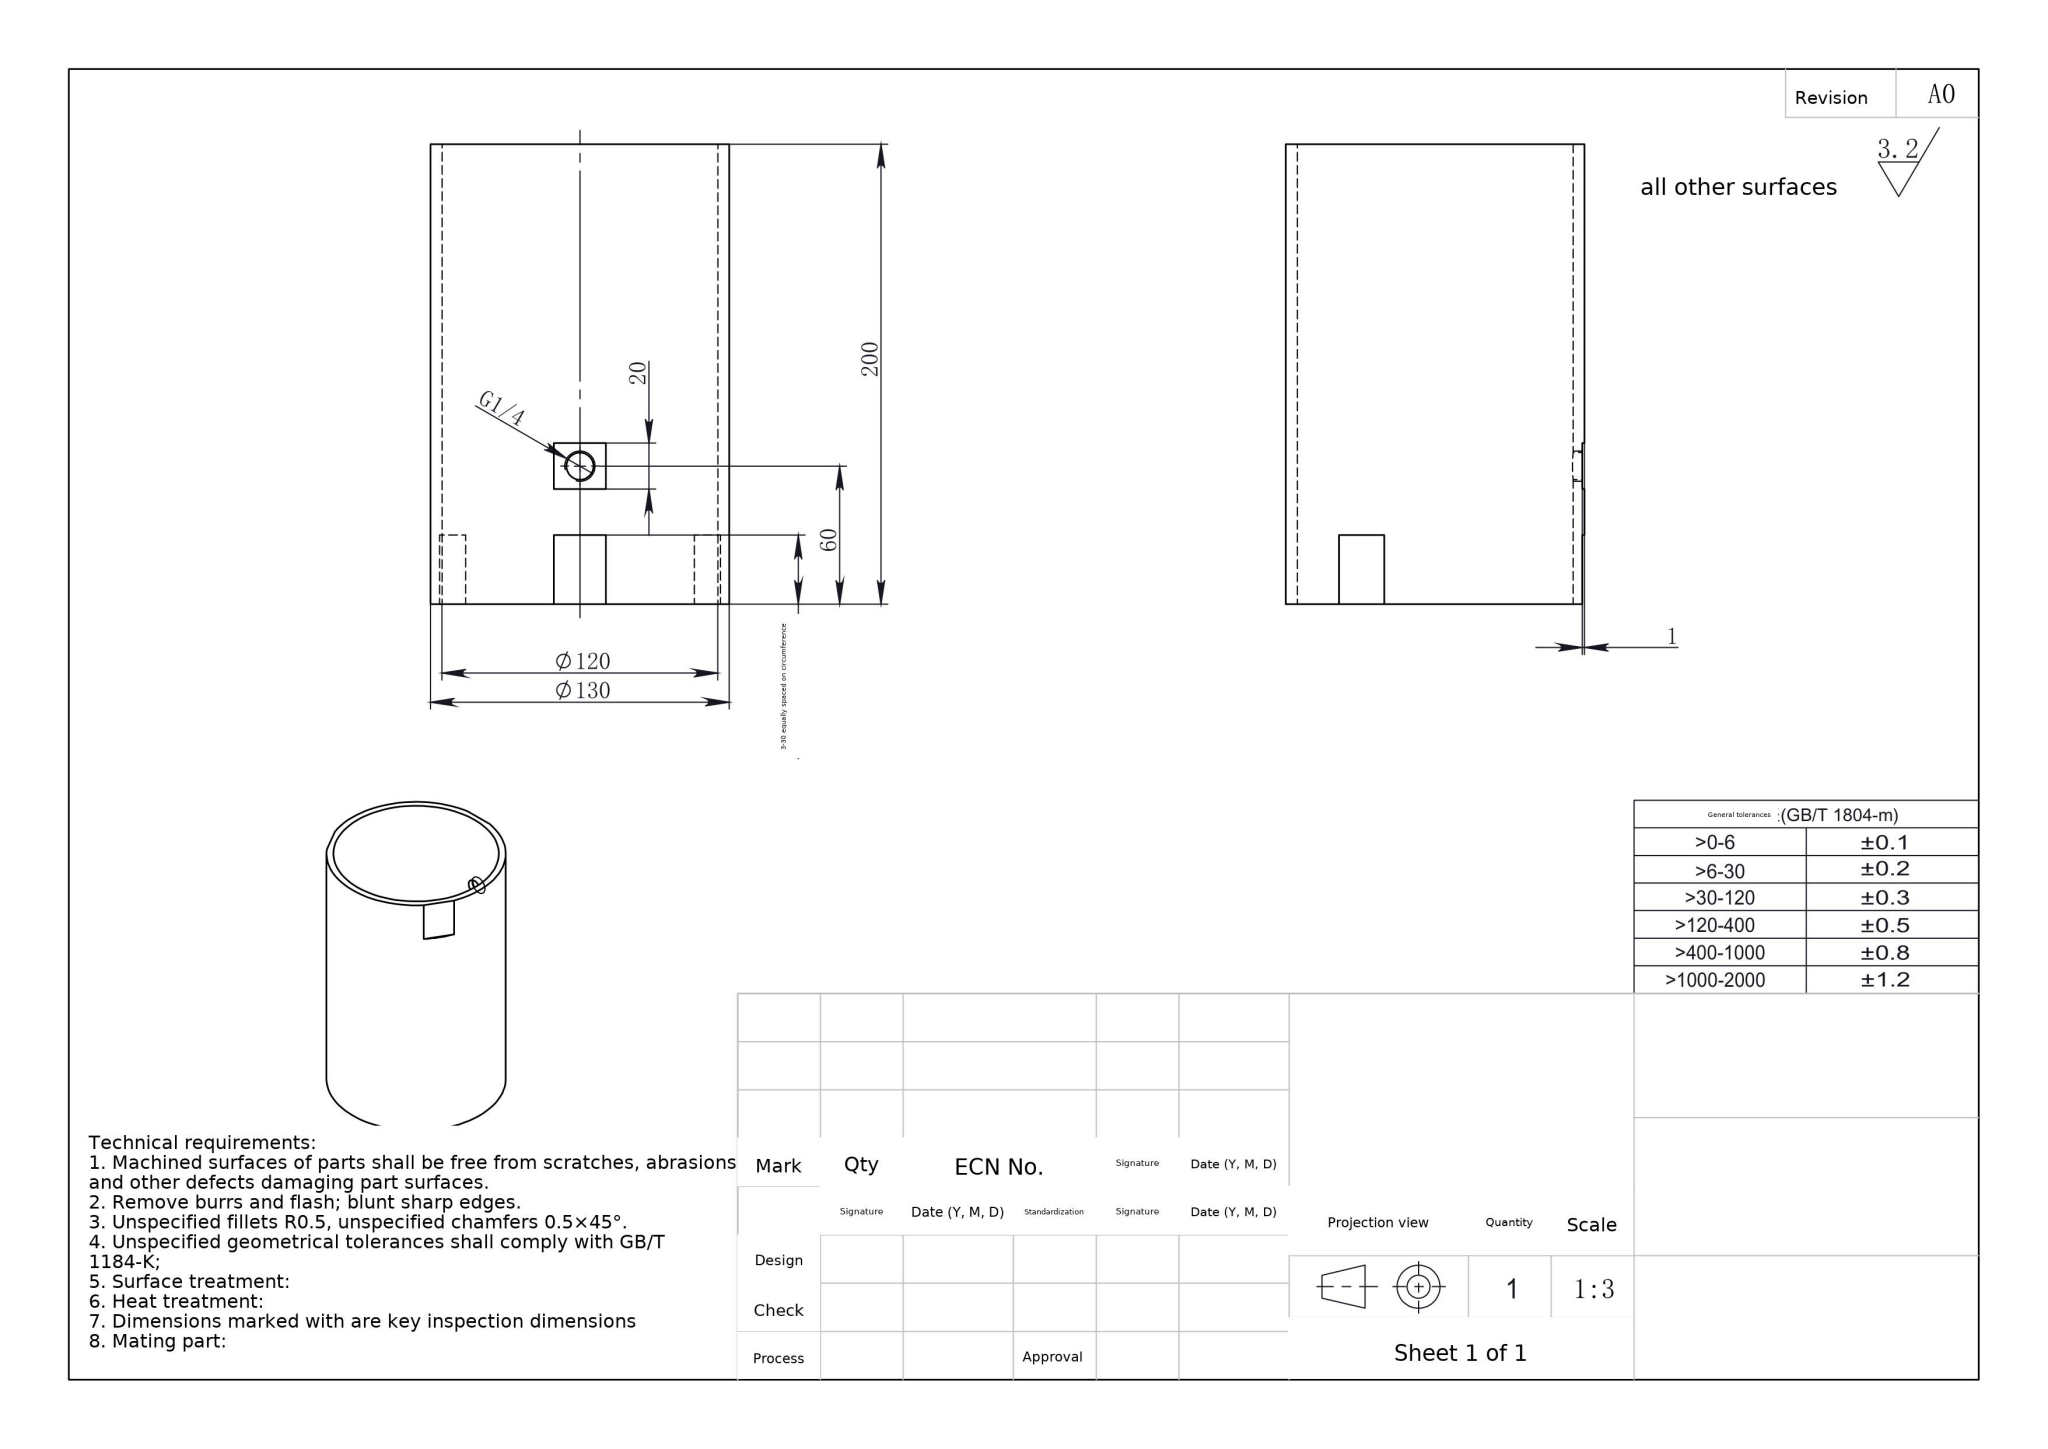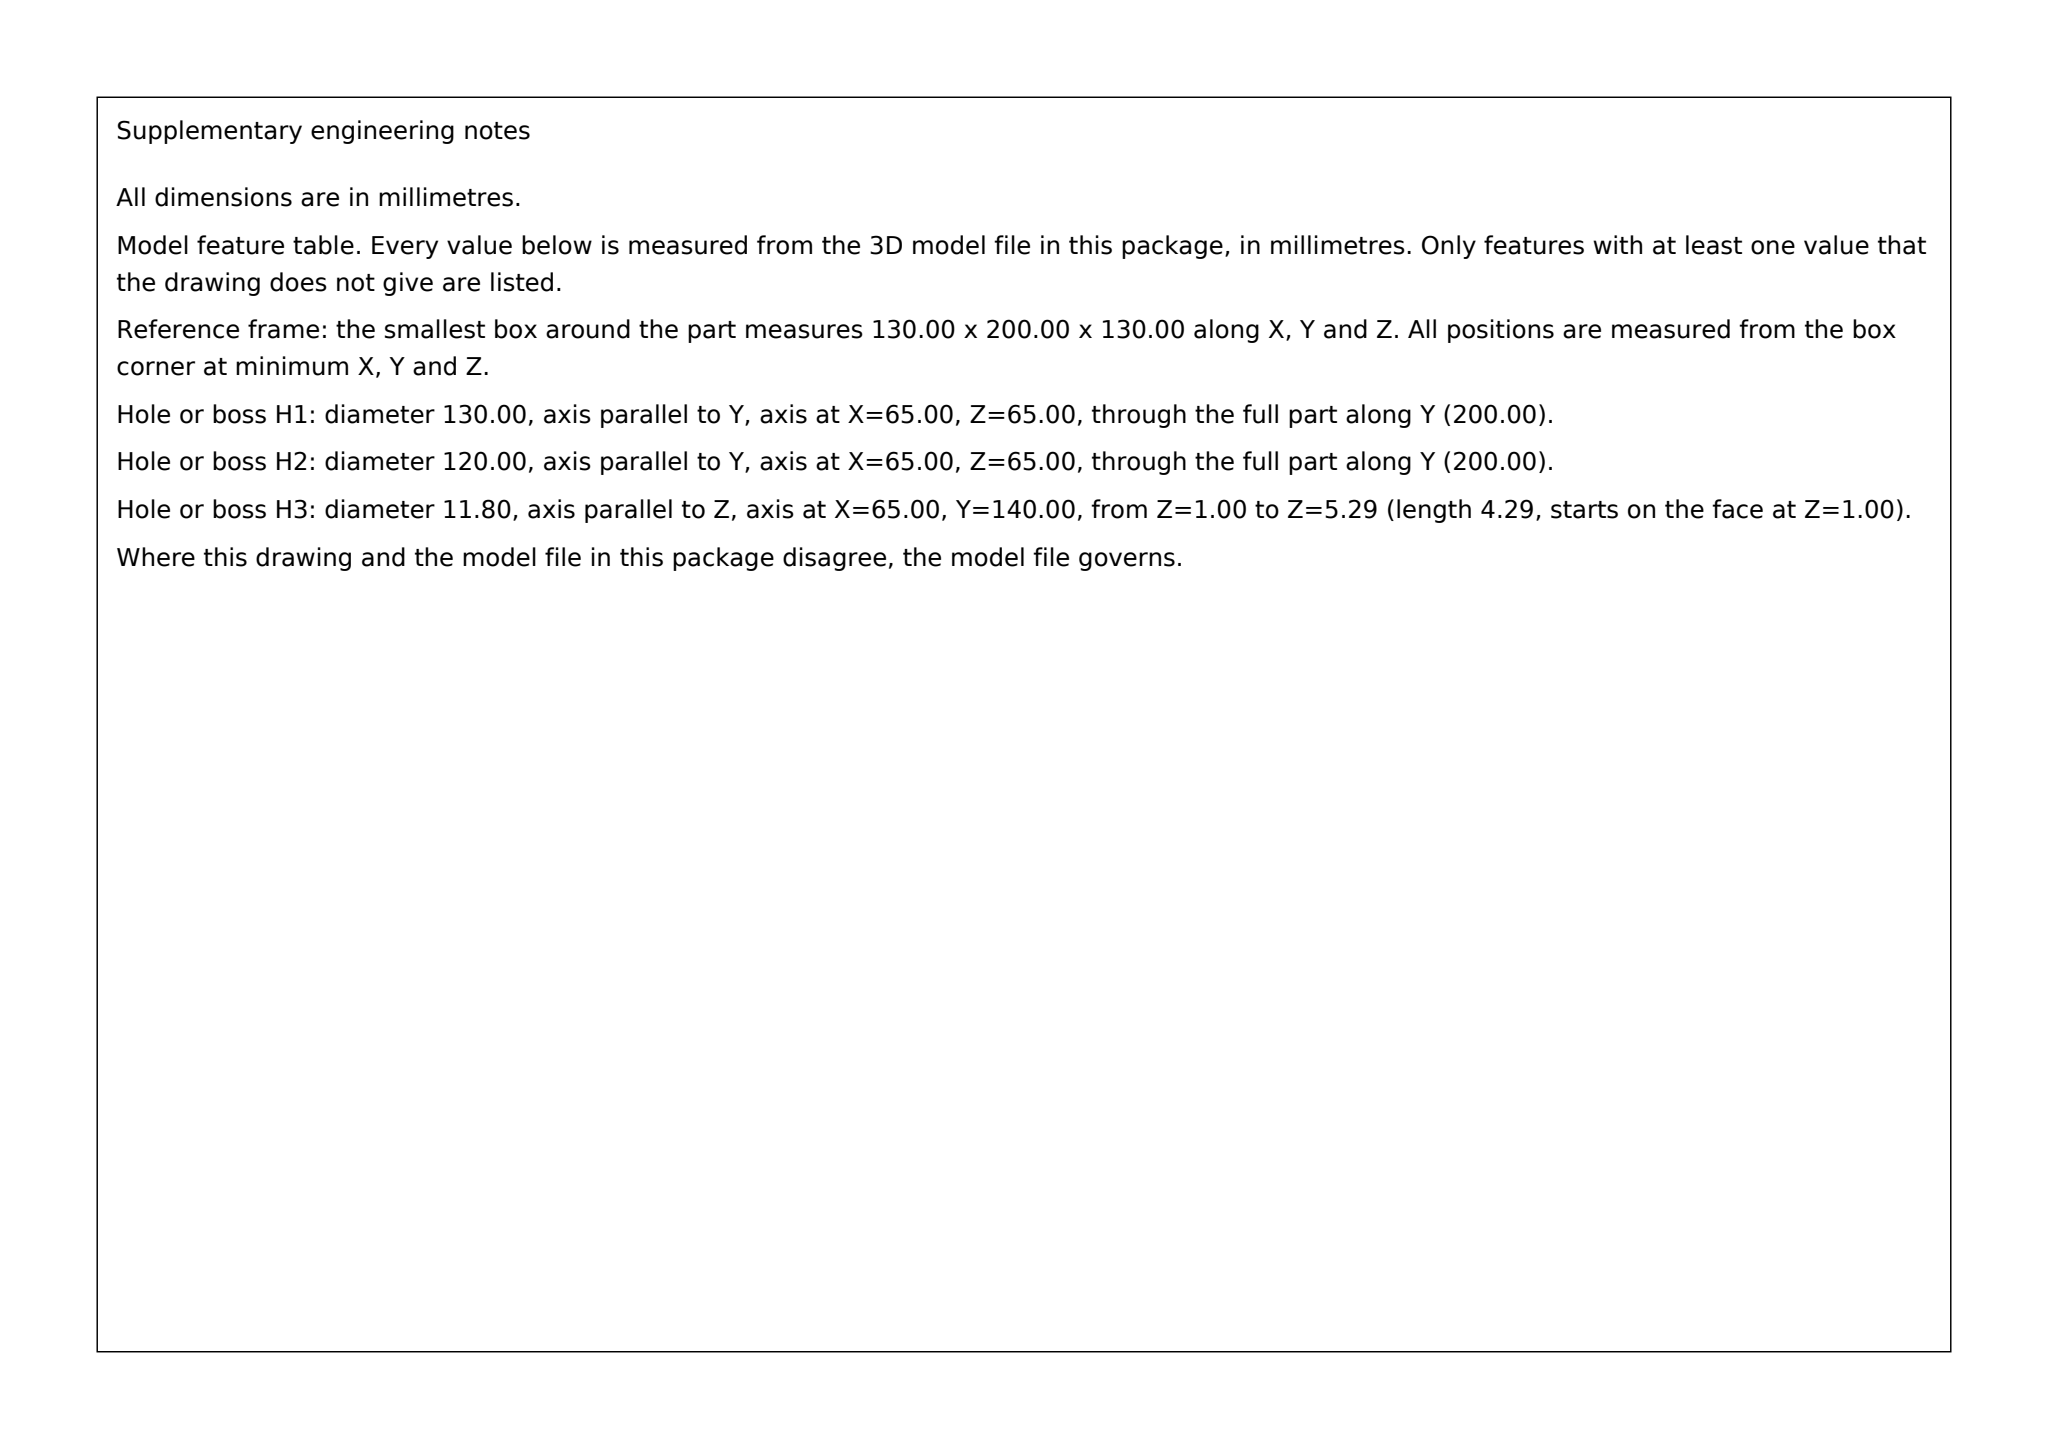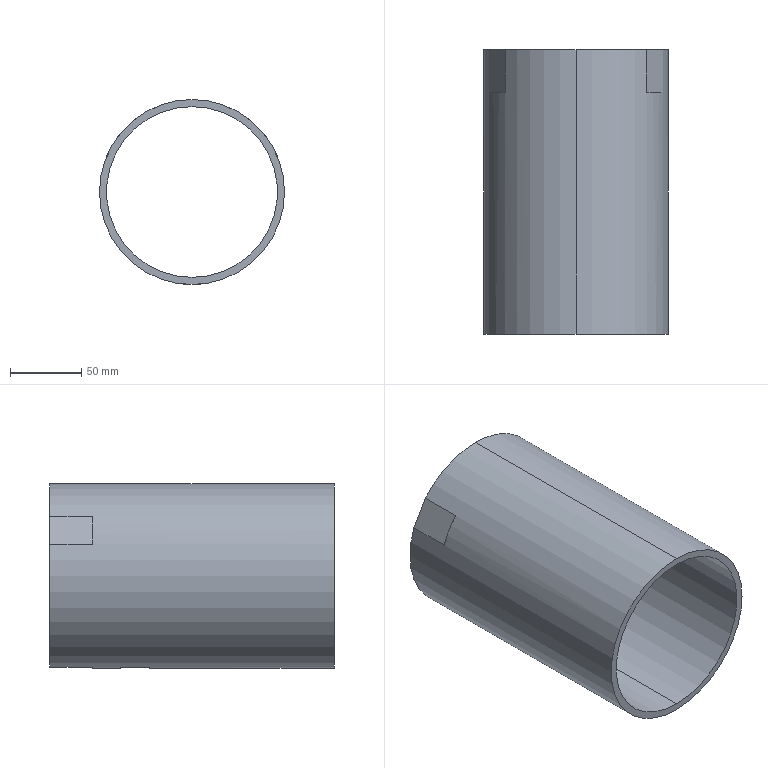Part | SolidWorks | mm | 1 solid | 17 faces | box 130 x 200 x 130 mm | volume 390585 mm3 | plane 11 | cylinder 6 | commonest cylinder face diameters 11.8 x2 120 x2 130 x2
build123d program:
from build123d import *

# Parameters (mm, degrees)
SKETCH1_R               = 65
SKETCH1_R_2             = 60
EXTRUDE1_DEPTH          = 200
SKETCH2_W               = 33.209
SKETCH2_H               = 3.332
EXTRUDE2_DEPTH          = 30
CIRPATTERN1_COUNT       = 3
SKETCH3_W               = 7.334
SKETCH3_H               = 20
EXTRUDE3_DEPTH          = 65
G1_4_TAPPED_HOLE1_D     = 11.8
G1_4_TAPPED_HOLE1_DEPTH = 30.32
G1_4_TAPPED_HOLE1_TIP   = 3.545


with BuildPart() as part:
    # Sketch1 → Extrude1 (new body)
    with BuildSketch(Plane(origin=(0, 0, 0), x_dir=(1, 0, 0), z_dir=(0, 1, 0))):
        with Locations(Location((0, 0, 0), (0, 0, 270))):
            Circle(SKETCH1_R)
        with Locations(Location((0, 0, 0), (0, 0, 270))):
            Circle(SKETCH1_R_2, mode=Mode.SUBTRACT)
    extrude(amount=EXTRUDE1_DEPTH)

    # Sketch2 → Extrude2 (cut)
    with BuildSketch(Plane(origin=(0, 200, 0), x_dir=(1, 0, 0), z_dir=(0, 1, 0))):
        with Locations((1.919, 65.666)):
            Rectangle(SKETCH2_W, SKETCH2_H)
    extrude2 = extrude(amount=-EXTRUDE2_DEPTH, mode=Mode.SUBTRACT)

    # CirPattern1: Extrude2 ×3 about axis
    cirpattern1_axis = Axis((0, 0, 0), (0, 1, 0))
    for i in range(1, CIRPATTERN1_COUNT):
        add(extrude2.rotate(cirpattern1_axis, i * 360 / CIRPATTERN1_COUNT), mode=Mode.SUBTRACT)

    # Sketch3 → Extrude3 (cut, symmetric)
    with BuildSketch(Plane(origin=(0, 0, 0), x_dir=(0, 0, -1), z_dir=(1, 0, 0))):
        with Locations((67.667, 140)):
            Rectangle(SKETCH3_W, SKETCH3_H)
    extrude(amount=EXTRUDE3_DEPTH, both=True, mode=Mode.SUBTRACT)

    # G1_4 Tapped Hole1
    with Locations(Plane(origin=(0, 0, -64), x_dir=(-1, 0, 0), z_dir=(0, 0, -1))):
        with Locations((0, 140)):
            Hole(G1_4_TAPPED_HOLE1_D / 2, depth=G1_4_TAPPED_HOLE1_DEPTH)
            with Locations((0, 0, -(G1_4_TAPPED_HOLE1_DEPTH + G1_4_TAPPED_HOLE1_TIP / 2))):  # 118° drill point
                Cone(0, G1_4_TAPPED_HOLE1_D / 2, G1_4_TAPPED_HOLE1_TIP, mode=Mode.SUBTRACT)


solid = part.part
STEP:
#1=CARTESIAN_POINT('',(0.,134.1,-60.));
#2=VERTEX_POINT('',#1);
#3=CARTESIAN_POINT('',(5.9,140.,-59.709));
#4=VERTEX_POINT('',#3);
#5=CARTESIAN_POINT('',(0.,134.1,-60.));
#6=CARTESIAN_POINT('',(0.3853,134.1,-60.));
#7=CARTESIAN_POINT('',(0.7684,134.137,-59.996));
#8=CARTESIAN_POINT('',(1.34,134.251,-59.985));
#9=CARTESIAN_POINT('',(1.529,134.298,-59.981));
#10=CARTESIAN_POINT('',(1.899,134.411,-59.97));
#11=CARTESIAN_POINT('',(2.261,134.54,-59.958));
#12=CARTESIAN_POINT('',(2.609,134.705,-59.943));
#13=CARTESIAN_POINT('',(2.95,134.887,-59.928));
#14=CARTESIAN_POINT('',(3.117,134.987,-59.919));
#15=CARTESIAN_POINT('',(3.601,135.311,-59.893));
#16=CARTESIAN_POINT('',(3.898,135.555,-59.874));
#17=CARTESIAN_POINT('',(4.443,136.099,-59.836));
#18=CARTESIAN_POINT('',(4.692,136.402,-59.817));
#19=CARTESIAN_POINT('',(5.12,137.044,-59.782));
#20=CARTESIAN_POINT('',(5.302,137.382,-59.765));
#21=CARTESIAN_POINT('',(5.524,137.918,-59.745));
#22=CARTESIAN_POINT('',(5.59,138.102,-59.739));
#23=CARTESIAN_POINT('',(5.702,138.473,-59.728));
#24=CARTESIAN_POINT('',(5.749,138.661,-59.724));
#25=CARTESIAN_POINT('',(5.862,139.227,-59.713));
#26=CARTESIAN_POINT('',(5.9,139.61,-59.709));
#27=CARTESIAN_POINT('',(5.9,140.,-59.709));
#28=B_SPLINE_CURVE_WITH_KNOTS('',3,(#5,#6,#7,#8,#9,#10,#11,#12,#13,#14,#15,#16,#17,#18,#19,#20,#21,#22,#23,#24,#25,#26,#27),.UNSPECIFIED.,.F.,.F.,(4,2,2,1,2,2,2,2,2,2,2,4),(0.01846,0.01961,0.02019,0.02076,0.02134,0.02192,0.02307,0.02423,0.02538,0.02596,0.02653,0.02769),.UNSPECIFIED.);
#29=EDGE_CURVE('',#2,#4,#28,.T.);
#30=ORIENTED_EDGE('',*,*,#29,.T.);
#31=CARTESIAN_POINT('',(5.9,140.,-64.));
#32=VERTEX_POINT('',#31);
#33=CARTESIAN_POINT('',(5.9,140.,-64.));
#34=DIRECTION('',(0.,0.,-1.));
#35=VECTOR('',#34,1000.);
#36=LINE('',#33,#35);
#37=EDGE_CURVE('',#4,#32,#36,.T.);
#38=ORIENTED_EDGE('',*,*,#37,.T.);
#39=CARTESIAN_POINT('',(-5.9,140.,-64.));
#40=VERTEX_POINT('',#39);
#41=CARTESIAN_POINT('',(0.,140.,-64.));
#42=DIRECTION('',(0.,0.,-1.));
#43=DIRECTION('',(-1.,0.,0.));
#44=AXIS2_PLACEMENT_3D('',#41,#42,#43);
#45=CIRCLE('',#44,5.9);
#46=EDGE_CURVE('',#32,#40,#45,.T.);
#47=ORIENTED_EDGE('',*,*,#46,.T.);
#48=CARTESIAN_POINT('',(-5.9,140.,-59.709));
#49=VERTEX_POINT('',#48);
#50=CARTESIAN_POINT('',(-5.9,140.,-64.));
#51=DIRECTION('',(0.,0.,-1.));
#52=VECTOR('',#51,1000.);
#53=LINE('',#50,#52);
#54=EDGE_CURVE('',#49,#40,#53,.T.);
#55=ORIENTED_EDGE('',*,*,#54,.F.);
#56=CARTESIAN_POINT('',(-5.9,140.,-59.709));
#57=CARTESIAN_POINT('',(-5.9,139.615,-59.709));
#58=CARTESIAN_POINT('',(-5.861,139.224,-59.713));
#59=CARTESIAN_POINT('',(-5.71,138.467,-59.728));
#60=CARTESIAN_POINT('',(-5.599,138.099,-59.738));
#61=CARTESIAN_POINT('',(-5.377,137.564,-59.759));
#62=CARTESIAN_POINT('',(-5.293,137.387,-59.766));
#63=CARTESIAN_POINT('',(-5.111,137.045,-59.782));
#64=CARTESIAN_POINT('',(-5.011,136.88,-59.79));
#65=CARTESIAN_POINT('',(-4.691,136.401,-59.817));
#66=CARTESIAN_POINT('',(-4.447,136.103,-59.836));
#67=CARTESIAN_POINT('',(-3.896,135.553,-59.874));
#68=CARTESIAN_POINT('',(-3.599,135.309,-59.893));
#69=CARTESIAN_POINT('',(-3.12,134.988,-59.919));
#70=CARTESIAN_POINT('',(-2.954,134.889,-59.927));
#71=CARTESIAN_POINT('',(-2.613,134.707,-59.943));
#72=CARTESIAN_POINT('',(-2.436,134.623,-59.951));
#73=CARTESIAN_POINT('',(-1.9,134.401,-59.971));
#74=CARTESIAN_POINT('',(-1.533,134.289,-59.982));
#75=CARTESIAN_POINT('',(-0.7762,134.139,-59.996));
#76=CARTESIAN_POINT('',(-0.3851,134.1,-60.));
#77=CARTESIAN_POINT('',(0.,134.1,-60.));
#78=B_SPLINE_CURVE_WITH_KNOTS('',3,(#56,#57,#58,#59,#60,#61,#62,#63,#64,#65,#66,#67,#68,#69,#70,#71,#72,#73,#74,#75,#76,#77),.UNSPECIFIED.,.F.,.F.,(4,2,2,2,2,2,2,2,2,2,4),(0.009231,0.01038,0.01154,0.01211,0.01269,0.01384,0.015,0.01557,0.01615,0.0173,0.01846),.UNSPECIFIED.);
#79=EDGE_CURVE('',#49,#2,#78,.T.);
#80=ORIENTED_EDGE('',*,*,#79,.T.);
#81=EDGE_LOOP('',(#30,#38,#47,#55,#80));
#82=FACE_OUTER_BOUND('',#81,.T.);
#83=CARTESIAN_POINT('',(0.,140.,-64.));
#84=DIRECTION('',(0.,0.,-1.));
#85=DIRECTION('',(-1.,0.,0.));
#86=AXIS2_PLACEMENT_3D('',#83,#84,#85);
#87=CYLINDRICAL_SURFACE('',#86,5.9);
#88=ADVANCED_FACE('',(#82),#87,.F.);
#89=CARTESIAN_POINT('',(0.,200.,-60.));
#90=VERTEX_POINT('',#89);
#91=CARTESIAN_POINT('',(0.,200.,60.));
#92=VERTEX_POINT('',#91);
#93=CARTESIAN_POINT('',(0.,200.,0.));
#94=DIRECTION('',(0.,1.,0.));
#95=DIRECTION('',(0.,0.,1.));
#96=AXIS2_PLACEMENT_3D('',#93,#94,#95);
#97=CIRCLE('',#96,60.);
#98=EDGE_CURVE('',#90,#92,#97,.T.);
#99=ORIENTED_EDGE('',*,*,#98,.T.);
#100=CARTESIAN_POINT('',(0.,0.,60.));
#101=VERTEX_POINT('',#100);
#102=CARTESIAN_POINT('',(0.,200.,60.));
#103=DIRECTION('',(0.,-1.,0.));
#104=VECTOR('',#103,1000.);
#105=LINE('',#102,#104);
#106=EDGE_CURVE('',#92,#101,#105,.T.);
#107=ORIENTED_EDGE('',*,*,#106,.T.);
#108=CARTESIAN_POINT('',(0.,0.,-60.));
#109=VERTEX_POINT('',#108);
#110=CARTESIAN_POINT('',(0.,0.,0.));
#111=DIRECTION('',(0.,1.,0.));
#112=DIRECTION('',(0.,0.,1.));
#113=AXIS2_PLACEMENT_3D('',#110,#111,#112);
#114=CIRCLE('',#113,60.);
#115=EDGE_CURVE('',#109,#101,#114,.T.);
#116=ORIENTED_EDGE('',*,*,#115,.F.);
#117=CARTESIAN_POINT('',(0.,200.,-60.));
#118=DIRECTION('',(0.,-1.,0.));
#119=VECTOR('',#118,1000.);
#120=LINE('',#117,#119);
#121=EDGE_CURVE('',#2,#109,#120,.T.);
#122=ORIENTED_EDGE('',*,*,#121,.F.);
#123=ORIENTED_EDGE('',*,*,#79,.F.);
#124=CARTESIAN_POINT('',(-0.,145.9,-60.));
#125=VERTEX_POINT('',#124);
#126=CARTESIAN_POINT('',(-0.,145.9,-60.));
#127=CARTESIAN_POINT('',(-0.3902,145.9,-60.));
#128=CARTESIAN_POINT('',(-0.7738,145.862,-59.996));
#129=CARTESIAN_POINT('',(-1.34,145.749,-59.985));
#130=CARTESIAN_POINT('',(-1.527,145.702,-59.981));
#131=CARTESIAN_POINT('',(-1.898,145.59,-59.97));
#132=CARTESIAN_POINT('',(-2.082,145.524,-59.964));
#133=CARTESIAN_POINT('',(-2.618,145.302,-59.944));
#134=CARTESIAN_POINT('',(-2.957,145.12,-59.928));
#135=CARTESIAN_POINT('',(-3.598,144.692,-59.893));
#136=CARTESIAN_POINT('',(-3.902,144.443,-59.874));
#137=CARTESIAN_POINT('',(-4.445,143.898,-59.836));
#138=CARTESIAN_POINT('',(-4.69,143.601,-59.817));
#139=CARTESIAN_POINT('',(-5.013,143.117,-59.79));
#140=CARTESIAN_POINT('',(-5.113,142.95,-59.782));
#141=CARTESIAN_POINT('',(-5.295,142.609,-59.766));
#142=CARTESIAN_POINT('',(-5.46,142.261,-59.751));
#143=CARTESIAN_POINT('',(-5.589,141.899,-59.739));
#144=CARTESIAN_POINT('',(-5.702,141.529,-59.729));
#145=CARTESIAN_POINT('',(-5.749,141.34,-59.724));
#146=CARTESIAN_POINT('',(-5.863,140.768,-59.713));
#147=CARTESIAN_POINT('',(-5.9,140.385,-59.709));
#148=CARTESIAN_POINT('',(-5.9,140.,-59.709));
#149=B_SPLINE_CURVE_WITH_KNOTS('',3,(#126,#127,#128,#129,#130,#131,#132,#133,#134,#135,#136,#137,#138,#139,#140,#141,#142,#143,#144,#145,#146,#147,#148),.UNSPECIFIED.,.F.,.F.,(4,2,2,2,2,2,2,2,1,2,2,4),(0.,0.001154,0.001731,0.002308,0.003462,0.004615,0.005769,0.006346,0.006923,0.0075,0.008077,0.009231),.UNSPECIFIED.);
#150=EDGE_CURVE('',#125,#49,#149,.T.);
#151=ORIENTED_EDGE('',*,*,#150,.F.);
#152=CARTESIAN_POINT('',(0.,200.,-60.));
#153=DIRECTION('',(0.,-1.,0.));
#154=VECTOR('',#153,1000.);
#155=LINE('',#152,#154);
#156=EDGE_CURVE('',#90,#125,#155,.T.);
#157=ORIENTED_EDGE('',*,*,#156,.F.);
#158=EDGE_LOOP('',(#99,#107,#116,#122,#123,#151,#157));
#159=FACE_OUTER_BOUND('',#158,.T.);
#160=CARTESIAN_POINT('',(0.,200.,0.));
#161=DIRECTION('',(0.,-1.,0.));
#162=DIRECTION('',(0.,0.,-1.));
#163=AXIS2_PLACEMENT_3D('',#160,#161,#162);
#164=CYLINDRICAL_SURFACE('',#163,60.);
#165=ADVANCED_FACE('',(#159),#164,.F.);
#166=CARTESIAN_POINT('',(0.,200.,65.));
#167=VERTEX_POINT('',#166);
#168=CARTESIAN_POINT('',(49.747,200.,41.836));
#169=VERTEX_POINT('',#168);
#170=CARTESIAN_POINT('',(0.,200.,0.));
#171=DIRECTION('',(0.,1.,0.));
#172=DIRECTION('',(0.,0.,1.));
#173=AXIS2_PLACEMENT_3D('',#170,#171,#172);
#174=CIRCLE('',#173,65.);
#175=EDGE_CURVE('',#167,#169,#174,.T.);
#176=ORIENTED_EDGE('',*,*,#175,.F.);
#177=CARTESIAN_POINT('',(0.,0.,65.));
#178=VERTEX_POINT('',#177);
#179=CARTESIAN_POINT('',(0.,200.,65.));
#180=DIRECTION('',(0.,-1.,0.));
#181=VECTOR('',#180,1000.);
#182=LINE('',#179,#181);
#183=EDGE_CURVE('',#167,#178,#182,.T.);
#184=ORIENTED_EDGE('',*,*,#183,.T.);
#185=CARTESIAN_POINT('',(0.,0.,-65.));
#186=VERTEX_POINT('',#185);
#187=CARTESIAN_POINT('',(0.,0.,0.));
#188=DIRECTION('',(0.,1.,0.));
#189=DIRECTION('',(0.,0.,1.));
#190=AXIS2_PLACEMENT_3D('',#187,#188,#189);
#191=CIRCLE('',#190,65.);
#192=EDGE_CURVE('',#178,#186,#191,.T.);
#193=ORIENTED_EDGE('',*,*,#192,.T.);
#194=CARTESIAN_POINT('',(0.,130.,-65.));
#195=VERTEX_POINT('',#194);
#196=CARTESIAN_POINT('',(0.,200.,-65.));
#197=DIRECTION('',(0.,-1.,0.));
#198=VECTOR('',#197,1000.);
#199=LINE('',#196,#198);
#200=EDGE_CURVE('',#195,#186,#199,.T.);
#201=ORIENTED_EDGE('',*,*,#200,.F.);
#202=CARTESIAN_POINT('',(11.358,130.,-64.));
#203=VERTEX_POINT('',#202);
#204=CARTESIAN_POINT('',(0.,130.,0.));
#205=DIRECTION('',(0.,-1.,0.));
#206=DIRECTION('',(0.,0.,-1.));
#207=AXIS2_PLACEMENT_3D('',#204,#205,#206);
#208=CIRCLE('',#207,65.);
#209=EDGE_CURVE('',#195,#203,#208,.T.);
#210=ORIENTED_EDGE('',*,*,#209,.T.);
#211=CARTESIAN_POINT('',(11.358,150.,-64.));
#212=VERTEX_POINT('',#211);
#213=CARTESIAN_POINT('',(11.358,200.,-64.));
#214=DIRECTION('',(0.,1.,0.));
#215=VECTOR('',#214,1000.);
#216=LINE('',#213,#215);
#217=EDGE_CURVE('',#203,#212,#216,.T.);
#218=ORIENTED_EDGE('',*,*,#217,.T.);
#219=CARTESIAN_POINT('',(0.,150.,-65.));
#220=VERTEX_POINT('',#219);
#221=CARTESIAN_POINT('',(0.,150.,0.));
#222=DIRECTION('',(0.,1.,0.));
#223=DIRECTION('',(0.,0.,1.));
#224=AXIS2_PLACEMENT_3D('',#221,#222,#223);
#225=CIRCLE('',#224,65.);
#226=EDGE_CURVE('',#212,#220,#225,.T.);
#227=ORIENTED_EDGE('',*,*,#226,.T.);
#228=CARTESIAN_POINT('',(0.,170.,-65.));
#229=VERTEX_POINT('',#228);
#230=CARTESIAN_POINT('',(0.,200.,-65.));
#231=DIRECTION('',(0.,-1.,0.));
#232=VECTOR('',#231,1000.);
#233=LINE('',#230,#232);
#234=EDGE_CURVE('',#229,#220,#233,.T.);
#235=ORIENTED_EDGE('',*,*,#234,.F.);
#236=CARTESIAN_POINT('',(11.358,170.,-64.));
#237=VERTEX_POINT('',#236);
#238=CARTESIAN_POINT('',(0.,170.,0.));
#239=DIRECTION('',(0.,1.,0.));
#240=DIRECTION('',(0.,0.,1.));
#241=AXIS2_PLACEMENT_3D('',#238,#239,#240);
#242=CIRCLE('',#241,65.);
#243=EDGE_CURVE('',#237,#229,#242,.T.);
#244=ORIENTED_EDGE('',*,*,#243,.F.);
#245=CARTESIAN_POINT('',(11.358,200.,-64.));
#246=VERTEX_POINT('',#245);
#247=CARTESIAN_POINT('',(11.358,200.,-64.));
#248=DIRECTION('',(0.,1.,0.));
#249=VECTOR('',#248,1000.);
#250=LINE('',#247,#249);
#251=EDGE_CURVE('',#237,#246,#250,.T.);
#252=ORIENTED_EDGE('',*,*,#251,.T.);
#253=CARTESIAN_POINT('',(61.105,200.,22.164));
#254=VERTEX_POINT('',#253);
#255=CARTESIAN_POINT('',(0.,200.,0.));
#256=DIRECTION('',(0.,1.,0.));
#257=DIRECTION('',(0.,0.,1.));
#258=AXIS2_PLACEMENT_3D('',#255,#256,#257);
#259=CIRCLE('',#258,65.);
#260=EDGE_CURVE('',#254,#246,#259,.T.);
#261=ORIENTED_EDGE('',*,*,#260,.F.);
#262=CARTESIAN_POINT('',(61.105,170.,22.164));
#263=VERTEX_POINT('',#262);
#264=CARTESIAN_POINT('',(61.105,200.,22.164));
#265=DIRECTION('',(0.,-1.,0.));
#266=VECTOR('',#265,1000.);
#267=LINE('',#264,#266);
#268=EDGE_CURVE('',#254,#263,#267,.T.);
#269=ORIENTED_EDGE('',*,*,#268,.T.);
#270=CARTESIAN_POINT('',(49.747,170.,41.836));
#271=VERTEX_POINT('',#270);
#272=CARTESIAN_POINT('',(0.,170.,0.));
#273=DIRECTION('',(0.,1.,0.));
#274=DIRECTION('',(0.,0.,1.));
#275=AXIS2_PLACEMENT_3D('',#272,#273,#274);
#276=CIRCLE('',#275,65.);
#277=EDGE_CURVE('',#271,#263,#276,.T.);
#278=ORIENTED_EDGE('',*,*,#277,.F.);
#279=CARTESIAN_POINT('',(49.747,200.,41.836));
#280=DIRECTION('',(0.,1.,0.));
#281=VECTOR('',#280,1000.);
#282=LINE('',#279,#281);
#283=EDGE_CURVE('',#271,#169,#282,.T.);
#284=ORIENTED_EDGE('',*,*,#283,.T.);
#285=EDGE_LOOP('',(#176,#184,#193,#201,#210,#218,#227,#235,#244,#252,#261,#269,#278,#284));
#286=FACE_OUTER_BOUND('',#285,.T.);
#287=CARTESIAN_POINT('',(0.,200.,0.));
#288=DIRECTION('',(0.,-1.,0.));
#289=DIRECTION('',(0.,0.,-1.));
#290=AXIS2_PLACEMENT_3D('',#287,#288,#289);
#291=CYLINDRICAL_SURFACE('',#290,65.);
#292=ADVANCED_FACE('',(#286),#291,.T.);
#293=CARTESIAN_POINT('',(-49.747,200.,41.836));
#294=VERTEX_POINT('',#293);
#295=CARTESIAN_POINT('',(-61.105,200.,22.164));
#296=VERTEX_POINT('',#295);
#297=CARTESIAN_POINT('',(-48.083,200.,44.718));
#298=DIRECTION('',(-0.5,0.,-0.866));
#299=VECTOR('',#298,1000.);
#300=LINE('',#297,#299);
#301=EDGE_CURVE('',#294,#296,#300,.T.);
#302=ORIENTED_EDGE('',*,*,#301,.F.);
#303=CARTESIAN_POINT('',(0.,200.,0.));
#304=DIRECTION('',(0.,1.,0.));
#305=DIRECTION('',(0.,0.,1.));
#306=AXIS2_PLACEMENT_3D('',#303,#304,#305);
#307=CIRCLE('',#306,65.);
#308=EDGE_CURVE('',#294,#167,#307,.T.);
#309=ORIENTED_EDGE('',*,*,#308,.T.);
#310=ORIENTED_EDGE('',*,*,#175,.T.);
#311=CARTESIAN_POINT('',(62.768,200.,19.282));
#312=DIRECTION('',(-0.5,0.,0.866));
#313=VECTOR('',#312,1000.);
#314=LINE('',#311,#313);
#315=EDGE_CURVE('',#254,#169,#314,.T.);
#316=ORIENTED_EDGE('',*,*,#315,.F.);
#317=ORIENTED_EDGE('',*,*,#260,.T.);
#318=CARTESIAN_POINT('',(-11.358,200.,-64.));
#319=VERTEX_POINT('',#318);
#320=CARTESIAN_POINT('',(-14.685,200.,-64.));
#321=DIRECTION('',(1.,0.,0.));
#322=VECTOR('',#321,1000.);
#323=LINE('',#320,#322);
#324=EDGE_CURVE('',#319,#246,#323,.T.);
#325=ORIENTED_EDGE('',*,*,#324,.F.);
#326=CARTESIAN_POINT('',(0.,200.,0.));
#327=DIRECTION('',(0.,1.,0.));
#328=DIRECTION('',(0.,0.,1.));
#329=AXIS2_PLACEMENT_3D('',#326,#327,#328);
#330=CIRCLE('',#329,65.);
#331=EDGE_CURVE('',#319,#296,#330,.T.);
#332=ORIENTED_EDGE('',*,*,#331,.T.);
#333=EDGE_LOOP('',(#302,#309,#310,#316,#317,#325,#332));
#334=FACE_OUTER_BOUND('',#333,.T.);
#335=ORIENTED_EDGE('',*,*,#98,.F.);
#336=CARTESIAN_POINT('',(0.,200.,0.));
#337=DIRECTION('',(0.,1.,0.));
#338=DIRECTION('',(0.,0.,1.));
#339=AXIS2_PLACEMENT_3D('',#336,#337,#338);
#340=CIRCLE('',#339,60.);
#341=EDGE_CURVE('',#92,#90,#340,.T.);
#342=ORIENTED_EDGE('',*,*,#341,.F.);
#343=EDGE_LOOP('',(#335,#342));
#344=FACE_BOUND('',#343,.T.);
#345=CARTESIAN_POINT('',(0.,200.,0.));
#346=DIRECTION('',(0.,1.,0.));
#347=DIRECTION('',(0.,0.,1.));
#348=AXIS2_PLACEMENT_3D('',#345,#346,#347);
#349=PLANE('',#348);
#350=ADVANCED_FACE('',(#334,#344),#349,.T.);
#351=CARTESIAN_POINT('',(0.,0.,0.));
#352=DIRECTION('',(0.,1.,0.));
#353=DIRECTION('',(0.,0.,1.));
#354=AXIS2_PLACEMENT_3D('',#351,#352,#353);
#355=CIRCLE('',#354,65.);
#356=EDGE_CURVE('',#186,#178,#355,.T.);
#357=ORIENTED_EDGE('',*,*,#356,.F.);
#358=ORIENTED_EDGE('',*,*,#192,.F.);
#359=EDGE_LOOP('',(#357,#358));
#360=FACE_OUTER_BOUND('',#359,.T.);
#361=ORIENTED_EDGE('',*,*,#115,.T.);
#362=CARTESIAN_POINT('',(0.,0.,0.));
#363=DIRECTION('',(0.,1.,0.));
#364=DIRECTION('',(0.,0.,1.));
#365=AXIS2_PLACEMENT_3D('',#362,#363,#364);
#366=CIRCLE('',#365,60.);
#367=EDGE_CURVE('',#101,#109,#366,.T.);
#368=ORIENTED_EDGE('',*,*,#367,.T.);
#369=EDGE_LOOP('',(#361,#368));
#370=FACE_BOUND('',#369,.T.);
#371=CARTESIAN_POINT('',(0.,0.,0.));
#372=DIRECTION('',(0.,1.,0.));
#373=DIRECTION('',(0.,0.,1.));
#374=AXIS2_PLACEMENT_3D('',#371,#372,#373);
#375=PLANE('',#374);
#376=ADVANCED_FACE('',(#360,#370),#375,.F.);
#377=ORIENTED_EDGE('',*,*,#183,.F.);
#378=ORIENTED_EDGE('',*,*,#308,.F.);
#379=CARTESIAN_POINT('',(-49.747,170.,41.836));
#380=VERTEX_POINT('',#379);
#381=CARTESIAN_POINT('',(-49.747,200.,41.836));
#382=DIRECTION('',(0.,-1.,0.));
#383=VECTOR('',#382,1000.);
#384=LINE('',#381,#383);
#385=EDGE_CURVE('',#294,#380,#384,.T.);
#386=ORIENTED_EDGE('',*,*,#385,.T.);
#387=CARTESIAN_POINT('',(-61.105,170.,22.164));
#388=VERTEX_POINT('',#387);
#389=CARTESIAN_POINT('',(0.,170.,0.));
#390=DIRECTION('',(0.,1.,0.));
#391=DIRECTION('',(0.,0.,1.));
#392=AXIS2_PLACEMENT_3D('',#389,#390,#391);
#393=CIRCLE('',#392,65.);
#394=EDGE_CURVE('',#388,#380,#393,.T.);
#395=ORIENTED_EDGE('',*,*,#394,.F.);
#396=CARTESIAN_POINT('',(-61.105,200.,22.164));
#397=DIRECTION('',(0.,1.,0.));
#398=VECTOR('',#397,1000.);
#399=LINE('',#396,#398);
#400=EDGE_CURVE('',#388,#296,#399,.T.);
#401=ORIENTED_EDGE('',*,*,#400,.T.);
#402=ORIENTED_EDGE('',*,*,#331,.F.);
#403=CARTESIAN_POINT('',(-11.358,170.,-64.));
#404=VERTEX_POINT('',#403);
#405=CARTESIAN_POINT('',(-11.358,200.,-64.));
#406=DIRECTION('',(0.,-1.,0.));
#407=VECTOR('',#406,1000.);
#408=LINE('',#405,#407);
#409=EDGE_CURVE('',#319,#404,#408,.T.);
#410=ORIENTED_EDGE('',*,*,#409,.T.);
#411=CARTESIAN_POINT('',(0.,170.,0.));
#412=DIRECTION('',(0.,1.,0.));
#413=DIRECTION('',(0.,0.,1.));
#414=AXIS2_PLACEMENT_3D('',#411,#412,#413);
#415=CIRCLE('',#414,65.);
#416=EDGE_CURVE('',#229,#404,#415,.T.);
#417=ORIENTED_EDGE('',*,*,#416,.F.);
#418=ORIENTED_EDGE('',*,*,#234,.T.);
#419=CARTESIAN_POINT('',(-11.358,150.,-64.));
#420=VERTEX_POINT('',#419);
#421=CARTESIAN_POINT('',(0.,150.,0.));
#422=DIRECTION('',(0.,1.,0.));
#423=DIRECTION('',(0.,0.,1.));
#424=AXIS2_PLACEMENT_3D('',#421,#422,#423);
#425=CIRCLE('',#424,65.);
#426=EDGE_CURVE('',#220,#420,#425,.T.);
#427=ORIENTED_EDGE('',*,*,#426,.T.);
#428=CARTESIAN_POINT('',(-11.358,130.,-64.));
#429=VERTEX_POINT('',#428);
#430=CARTESIAN_POINT('',(-11.358,200.,-64.));
#431=DIRECTION('',(0.,-1.,0.));
#432=VECTOR('',#431,1000.);
#433=LINE('',#430,#432);
#434=EDGE_CURVE('',#420,#429,#433,.T.);
#435=ORIENTED_EDGE('',*,*,#434,.T.);
#436=CARTESIAN_POINT('',(0.,130.,0.));
#437=DIRECTION('',(0.,-1.,0.));
#438=DIRECTION('',(0.,0.,-1.));
#439=AXIS2_PLACEMENT_3D('',#436,#437,#438);
#440=CIRCLE('',#439,65.);
#441=EDGE_CURVE('',#429,#195,#440,.T.);
#442=ORIENTED_EDGE('',*,*,#441,.T.);
#443=ORIENTED_EDGE('',*,*,#200,.T.);
#444=ORIENTED_EDGE('',*,*,#356,.T.);
#445=EDGE_LOOP('',(#377,#378,#386,#395,#401,#402,#410,#417,#418,#427,#435,#442,#443,#444));
#446=FACE_OUTER_BOUND('',#445,.T.);
#447=CARTESIAN_POINT('',(0.,200.,0.));
#448=DIRECTION('',(0.,-1.,0.));
#449=DIRECTION('',(0.,0.,-1.));
#450=AXIS2_PLACEMENT_3D('',#447,#448,#449);
#451=CYLINDRICAL_SURFACE('',#450,65.);
#452=ADVANCED_FACE('',(#446),#451,.T.);
#453=ORIENTED_EDGE('',*,*,#106,.F.);
#454=ORIENTED_EDGE('',*,*,#341,.T.);
#455=ORIENTED_EDGE('',*,*,#156,.T.);
#456=CARTESIAN_POINT('',(5.9,140.,-59.709));
#457=CARTESIAN_POINT('',(5.9,140.39,-59.709));
#458=CARTESIAN_POINT('',(5.862,140.773,-59.713));
#459=CARTESIAN_POINT('',(5.749,141.339,-59.724));
#460=CARTESIAN_POINT('',(5.703,141.526,-59.728));
#461=CARTESIAN_POINT('',(5.59,141.896,-59.739));
#462=CARTESIAN_POINT('',(5.525,142.08,-59.745));
#463=CARTESIAN_POINT('',(5.303,142.616,-59.765));
#464=CARTESIAN_POINT('',(5.121,142.955,-59.781));
#465=CARTESIAN_POINT('',(4.694,143.595,-59.817));
#466=CARTESIAN_POINT('',(4.445,143.899,-59.836));
#467=CARTESIAN_POINT('',(3.901,144.443,-59.874));
#468=CARTESIAN_POINT('',(3.605,144.687,-59.892));
#469=CARTESIAN_POINT('',(3.122,145.01,-59.919));
#470=CARTESIAN_POINT('',(2.955,145.111,-59.927));
#471=CARTESIAN_POINT('',(2.614,145.293,-59.943));
#472=CARTESIAN_POINT('',(2.441,145.375,-59.951));
#473=CARTESIAN_POINT('',(1.909,145.596,-59.971));
#474=CARTESIAN_POINT('',(1.538,145.709,-59.982));
#475=CARTESIAN_POINT('',(0.7753,145.862,-59.996));
#476=CARTESIAN_POINT('',(0.3898,145.9,-60.));
#477=CARTESIAN_POINT('',(-0.,145.9,-60.));
#478=B_SPLINE_CURVE_WITH_KNOTS('',3,(#456,#457,#458,#459,#460,#461,#462,#463,#464,#465,#466,#467,#468,#469,#470,#471,#472,#473,#474,#475,#476,#477),.UNSPECIFIED.,.F.,.F.,(4,2,2,2,2,2,2,2,2,2,4),(0.02769,0.02884,0.02942,0.02999,0.03115,0.0323,0.03345,0.03403,0.0346,0.03576,0.03691),.UNSPECIFIED.);
#479=EDGE_CURVE('',#4,#125,#478,.T.);
#480=ORIENTED_EDGE('',*,*,#479,.F.);
#481=ORIENTED_EDGE('',*,*,#29,.F.);
#482=ORIENTED_EDGE('',*,*,#121,.T.);
#483=ORIENTED_EDGE('',*,*,#367,.F.);
#484=EDGE_LOOP('',(#453,#454,#455,#480,#481,#482,#483));
#485=FACE_OUTER_BOUND('',#484,.T.);
#486=CARTESIAN_POINT('',(0.,200.,0.));
#487=DIRECTION('',(0.,-1.,0.));
#488=DIRECTION('',(0.,0.,-1.));
#489=AXIS2_PLACEMENT_3D('',#486,#487,#488);
#490=CYLINDRICAL_SURFACE('',#489,60.);
#491=ADVANCED_FACE('',(#485),#490,.F.);
#492=ORIENTED_EDGE('',*,*,#324,.T.);
#493=ORIENTED_EDGE('',*,*,#251,.F.);
#494=CARTESIAN_POINT('',(-14.685,170.,-64.));
#495=DIRECTION('',(1.,0.,0.));
#496=VECTOR('',#495,1000.);
#497=LINE('',#494,#496);
#498=EDGE_CURVE('',#404,#237,#497,.T.);
#499=ORIENTED_EDGE('',*,*,#498,.F.);
#500=ORIENTED_EDGE('',*,*,#409,.F.);
#501=EDGE_LOOP('',(#492,#493,#499,#500));
#502=FACE_OUTER_BOUND('',#501,.T.);
#503=CARTESIAN_POINT('',(-14.685,170.,-64.));
#504=DIRECTION('',(0.,0.,1.));
#505=DIRECTION('',(1.,0.,0.));
#506=AXIS2_PLACEMENT_3D('',#503,#504,#505);
#507=PLANE('',#506);
#508=ADVANCED_FACE('',(#502),#507,.F.);
#509=ORIENTED_EDGE('',*,*,#243,.T.);
#510=ORIENTED_EDGE('',*,*,#416,.T.);
#511=ORIENTED_EDGE('',*,*,#498,.T.);
#512=EDGE_LOOP('',(#509,#510,#511));
#513=FACE_OUTER_BOUND('',#512,.T.);
#514=CARTESIAN_POINT('',(0.,170.,0.));
#515=DIRECTION('',(0.,1.,0.));
#516=DIRECTION('',(0.,0.,1.));
#517=AXIS2_PLACEMENT_3D('',#514,#515,#516);
#518=PLANE('',#517);
#519=ADVANCED_FACE('',(#513),#518,.T.);
#520=ORIENTED_EDGE('',*,*,#315,.T.);
#521=ORIENTED_EDGE('',*,*,#283,.F.);
#522=CARTESIAN_POINT('',(62.768,170.,19.282));
#523=DIRECTION('',(-0.5,0.,0.866));
#524=VECTOR('',#523,1000.);
#525=LINE('',#522,#524);
#526=EDGE_CURVE('',#263,#271,#525,.T.);
#527=ORIENTED_EDGE('',*,*,#526,.F.);
#528=ORIENTED_EDGE('',*,*,#268,.F.);
#529=EDGE_LOOP('',(#520,#521,#527,#528));
#530=FACE_OUTER_BOUND('',#529,.T.);
#531=CARTESIAN_POINT('',(62.768,170.,19.282));
#532=DIRECTION('',(-0.866,0.,-0.5));
#533=DIRECTION('',(-0.5,0.,0.866));
#534=AXIS2_PLACEMENT_3D('',#531,#532,#533);
#535=PLANE('',#534);
#536=ADVANCED_FACE('',(#530),#535,.F.);
#537=ORIENTED_EDGE('',*,*,#277,.T.);
#538=ORIENTED_EDGE('',*,*,#526,.T.);
#539=EDGE_LOOP('',(#537,#538));
#540=FACE_OUTER_BOUND('',#539,.T.);
#541=CARTESIAN_POINT('',(0.,170.,0.));
#542=DIRECTION('',(0.,1.,0.));
#543=DIRECTION('',(-0.866,0.,-0.5));
#544=AXIS2_PLACEMENT_3D('',#541,#542,#543);
#545=PLANE('',#544);
#546=ADVANCED_FACE('',(#540),#545,.T.);
#547=ORIENTED_EDGE('',*,*,#301,.T.);
#548=ORIENTED_EDGE('',*,*,#400,.F.);
#549=CARTESIAN_POINT('',(-48.083,170.,44.718));
#550=DIRECTION('',(-0.5,0.,-0.866));
#551=VECTOR('',#550,1000.);
#552=LINE('',#549,#551);
#553=EDGE_CURVE('',#380,#388,#552,.T.);
#554=ORIENTED_EDGE('',*,*,#553,.F.);
#555=ORIENTED_EDGE('',*,*,#385,.F.);
#556=EDGE_LOOP('',(#547,#548,#554,#555));
#557=FACE_OUTER_BOUND('',#556,.T.);
#558=CARTESIAN_POINT('',(-48.083,170.,44.718));
#559=DIRECTION('',(0.866,0.,-0.5));
#560=DIRECTION('',(-0.5,0.,-0.866));
#561=AXIS2_PLACEMENT_3D('',#558,#559,#560);
#562=PLANE('',#561);
#563=ADVANCED_FACE('',(#557),#562,.F.);
#564=ORIENTED_EDGE('',*,*,#394,.T.);
#565=ORIENTED_EDGE('',*,*,#553,.T.);
#566=EDGE_LOOP('',(#564,#565));
#567=FACE_OUTER_BOUND('',#566,.T.);
#568=CARTESIAN_POINT('',(0.,170.,0.));
#569=DIRECTION('',(0.,1.,0.));
#570=DIRECTION('',(0.866,0.,-0.5));
#571=AXIS2_PLACEMENT_3D('',#568,#569,#570);
#572=PLANE('',#571);
#573=ADVANCED_FACE('',(#567),#572,.T.);
#574=CARTESIAN_POINT('',(-65.,130.,-64.));
#575=DIRECTION('',(1.,0.,0.));
#576=VECTOR('',#575,1000.);
#577=LINE('',#574,#576);
#578=EDGE_CURVE('',#429,#203,#577,.T.);
#579=ORIENTED_EDGE('',*,*,#578,.T.);
#580=ORIENTED_EDGE('',*,*,#209,.F.);
#581=ORIENTED_EDGE('',*,*,#441,.F.);
#582=EDGE_LOOP('',(#579,#580,#581));
#583=FACE_OUTER_BOUND('',#582,.T.);
#584=CARTESIAN_POINT('',(-65.,130.,-71.334));
#585=DIRECTION('',(0.,-1.,0.));
#586=DIRECTION('',(0.,0.,-1.));
#587=AXIS2_PLACEMENT_3D('',#584,#585,#586);
#588=PLANE('',#587);
#589=ADVANCED_FACE('',(#583),#588,.F.);
#590=CARTESIAN_POINT('',(0.,140.,-64.));
#591=DIRECTION('',(0.,0.,-1.));
#592=DIRECTION('',(-1.,0.,0.));
#593=AXIS2_PLACEMENT_3D('',#590,#591,#592);
#594=CIRCLE('',#593,5.9);
#595=EDGE_CURVE('',#40,#32,#594,.T.);
#596=ORIENTED_EDGE('',*,*,#595,.F.);
#597=ORIENTED_EDGE('',*,*,#46,.F.);
#598=EDGE_LOOP('',(#596,#597));
#599=FACE_BOUND('',#598,.T.);
#600=CARTESIAN_POINT('',(-65.,150.,-64.));
#601=DIRECTION('',(1.,0.,0.));
#602=VECTOR('',#601,1000.);
#603=LINE('',#600,#602);
#604=EDGE_CURVE('',#420,#212,#603,.T.);
#605=ORIENTED_EDGE('',*,*,#604,.T.);
#606=ORIENTED_EDGE('',*,*,#217,.F.);
#607=ORIENTED_EDGE('',*,*,#578,.F.);
#608=ORIENTED_EDGE('',*,*,#434,.F.);
#609=EDGE_LOOP('',(#605,#606,#607,#608));
#610=FACE_OUTER_BOUND('',#609,.T.);
#611=CARTESIAN_POINT('',(-65.,150.,-64.));
#612=DIRECTION('',(0.,0.,1.));
#613=DIRECTION('',(1.,0.,0.));
#614=AXIS2_PLACEMENT_3D('',#611,#612,#613);
#615=PLANE('',#614);
#616=ADVANCED_FACE('',(#599,#610),#615,.F.);
#617=ORIENTED_EDGE('',*,*,#604,.F.);
#618=ORIENTED_EDGE('',*,*,#426,.F.);
#619=ORIENTED_EDGE('',*,*,#226,.F.);
#620=EDGE_LOOP('',(#617,#618,#619));
#621=FACE_OUTER_BOUND('',#620,.T.);
#622=CARTESIAN_POINT('',(-65.,150.,-71.334));
#623=DIRECTION('',(0.,1.,0.));
#624=DIRECTION('',(0.,0.,1.));
#625=AXIS2_PLACEMENT_3D('',#622,#623,#624);
#626=PLANE('',#625);
#627=ADVANCED_FACE('',(#621),#626,.F.);
#628=ORIENTED_EDGE('',*,*,#37,.F.);
#629=ORIENTED_EDGE('',*,*,#479,.T.);
#630=ORIENTED_EDGE('',*,*,#150,.T.);
#631=ORIENTED_EDGE('',*,*,#54,.T.);
#632=ORIENTED_EDGE('',*,*,#595,.T.);
#633=EDGE_LOOP('',(#628,#629,#630,#631,#632));
#634=FACE_OUTER_BOUND('',#633,.T.);
#635=CARTESIAN_POINT('',(0.,140.,-64.));
#636=DIRECTION('',(0.,0.,-1.));
#637=DIRECTION('',(-1.,0.,0.));
#638=AXIS2_PLACEMENT_3D('',#635,#636,#637);
#639=CYLINDRICAL_SURFACE('',#638,5.9);
#640=ADVANCED_FACE('',(#634),#639,.F.);
#641=CLOSED_SHELL('',(#88,#165,#292,#350,#376,#452,#491,#508,#519,#536,#546,#563,#573,#589,#616,#627,#640));
#642=MANIFOLD_SOLID_BREP('',#641);
#643=CARTESIAN_POINT('',(0.,0.,0.));
#644=DIRECTION('',(0.,0.,1.));
#645=DIRECTION('',(1.,0.,0.));
#646=AXIS2_PLACEMENT_3D('',#643,#644,#645);
#647=(LENGTH_UNIT()NAMED_UNIT(*)SI_UNIT(.MILLI.,.METRE.));
#648=UNCERTAINTY_MEASURE_WITH_UNIT(LENGTH_MEASURE(0.00001),#647,'','');
#649=(NAMED_UNIT(*)PLANE_ANGLE_UNIT()SI_UNIT($,.RADIAN.));
#650=(NAMED_UNIT(*)SI_UNIT($,.STERADIAN.)SOLID_ANGLE_UNIT());
#651=(GEOMETRIC_REPRESENTATION_CONTEXT(3)GLOBAL_UNCERTAINTY_ASSIGNED_CONTEXT((#648))GLOBAL_UNIT_ASSIGNED_CONTEXT((#647,#649,#650))REPRESENTATION_CONTEXT('',''));
#652=ADVANCED_BREP_SHAPE_REPRESENTATION('',(#642,#646),#651);